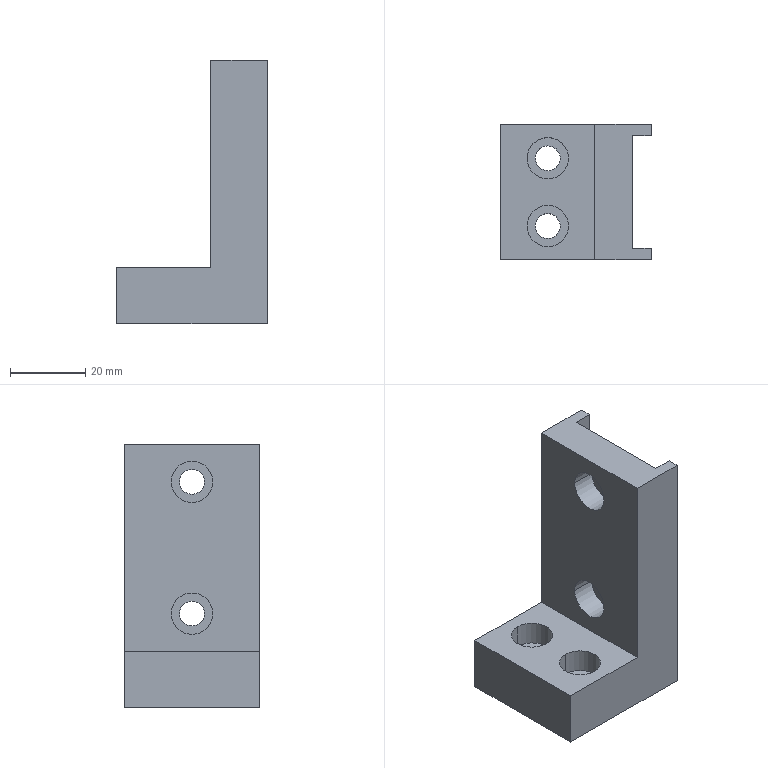Component | SolidWorks | XM-WST05-2008-2 | 1 solid | 32 faces | box 40 x 36 x 70 mm | volume 37532 mm3 | cylinder 16 | plane 16 | commonest cylinder face diameters 11 x8 6.6 x8
build123d program:
from build123d import *

# Parameters (mm, degrees)
BOSS_EXTRUDE1_DEPTH                             = 36
SKETCH2_W                                       = 10
SKETCH2_H                                       = 30
CUT_EXTRUDE1_DEPTH                              = 89.295
M6_HEX_SOCKET_HEAD_CAP_SCREW_CBORE1_D           = 6.6
M6_HEX_SOCKET_HEAD_CAP_SCREW_CBORE1_CBORE_D     = 11
M6_HEX_SOCKET_HEAD_CAP_SCREW_CBORE1_CBORE_DEPTH = 6.4
M6_HEX_SOCKET_HEAD_CAP_SCREW_CBORE2_D           = 6.6
M6_HEX_SOCKET_HEAD_CAP_SCREW_CBORE2_CBORE_D     = 11
M6_HEX_SOCKET_HEAD_CAP_SCREW_CBORE2_CBORE_DEPTH = 6.4


with BuildPart() as part:
    # Sketch1 → Boss-Extrude1 (new body)
    with BuildSketch(Plane.XY):
        Polygon((0, 0), (40, 0), (40, 15), (15, 15), (15, 70), (0, 70), align=None)
    extrude(amount=BOSS_EXTRUDE1_DEPTH)

    # Sketch2 → Cut-Extrude1 (cut, through all)
    with BuildSketch(Plane(origin=(0, 70, 0), x_dir=(1, 0, 0), z_dir=(0, 1, 0))):
        with Locations((0, -18)):
            Rectangle(SKETCH2_W, SKETCH2_H)
    extrude(amount=-CUT_EXTRUDE1_DEPTH, mode=Mode.SUBTRACT)

    # M6 Hex Socket Head Cap Screw CBORE1 (through all)
    with Locations(Plane(origin=(15, 0, 0), x_dir=(0, 0, -1), z_dir=(1, 0, 0))):
        with Locations((-18, 60), (-18, 25)):
            CounterBoreHole(M6_HEX_SOCKET_HEAD_CAP_SCREW_CBORE1_D / 2, M6_HEX_SOCKET_HEAD_CAP_SCREW_CBORE1_CBORE_D / 2, M6_HEX_SOCKET_HEAD_CAP_SCREW_CBORE1_CBORE_DEPTH)

    # M6 Hex Socket Head Cap Screw CBORE2 (through all)
    with Locations(Plane(origin=(0, 15, 0), x_dir=(-1, 0, 0), z_dir=(0, 1, 0))):
        with Locations((-27.5, 9), (-27.5, 27)):
            CounterBoreHole(M6_HEX_SOCKET_HEAD_CAP_SCREW_CBORE2_D / 2, M6_HEX_SOCKET_HEAD_CAP_SCREW_CBORE2_CBORE_D / 2, M6_HEX_SOCKET_HEAD_CAP_SCREW_CBORE2_CBORE_DEPTH)


solid = part.part

# Placed as in the assembly
solid = solid.moved(Location((-164.071, 30.669, 100.899), (-90, 0, 180)))
STEP:
#1=COLOUR_RGB('',0.7922,0.8196,0.9333);
#2=FILL_AREA_STYLE_COLOUR('',#1);
#3=FILL_AREA_STYLE('',(#2));
#4=SURFACE_STYLE_FILL_AREA(#3);
#5=SURFACE_SIDE_STYLE('',(#4));
#6=SURFACE_STYLE_USAGE(.BOTH.,#5);
#7=PRESENTATION_STYLE_ASSIGNMENT((#6));
#8=CARTESIAN_POINT('',(-7.542,1.345,4.311));
#9=VERTEX_POINT('',#8);
#10=CARTESIAN_POINT('',(-7.542,1.778,4.311));
#11=VERTEX_POINT('',#10);
#12=CARTESIAN_POINT('',(-7.542,1.562,4.311));
#13=DIRECTION('',(0.,-0.,1.));
#14=DIRECTION('',(0.,1.,0.));
#15=AXIS2_PLACEMENT_3D('',#12,#13,#14);
#16=CIRCLE('',#15,0.2165);
#17=EDGE_CURVE('',#9,#11,#16,.T.);
#18=ORIENTED_EDGE('',*,*,#17,.F.);
#19=CARTESIAN_POINT('',(-7.542,1.345,4.563));
#20=VERTEX_POINT('',#19);
#21=CARTESIAN_POINT('',(-7.542,1.345,4.563));
#22=DIRECTION('',(0.,-0.,1.));
#23=VECTOR('',#22,39.37);
#24=LINE('',#21,#23);
#25=EDGE_CURVE('',#9,#20,#24,.T.);
#26=ORIENTED_EDGE('',*,*,#25,.T.);
#27=CARTESIAN_POINT('',(-7.542,1.778,4.563));
#28=VERTEX_POINT('',#27);
#29=CARTESIAN_POINT('',(-7.542,1.562,4.563));
#30=DIRECTION('',(0.,-0.,1.));
#31=DIRECTION('',(0.,1.,0.));
#32=AXIS2_PLACEMENT_3D('',#29,#30,#31);
#33=CIRCLE('',#32,0.2165);
#34=EDGE_CURVE('',#20,#28,#33,.T.);
#35=ORIENTED_EDGE('',*,*,#34,.T.);
#36=CARTESIAN_POINT('',(-7.542,1.778,4.563));
#37=DIRECTION('',(0.,-0.,1.));
#38=VECTOR('',#37,39.37);
#39=LINE('',#36,#38);
#40=EDGE_CURVE('',#11,#28,#39,.T.);
#41=ORIENTED_EDGE('',*,*,#40,.F.);
#42=EDGE_LOOP('',(#18,#26,#35,#41));
#43=FACE_OUTER_BOUND('',#42,.T.);
#44=CARTESIAN_POINT('',(-7.542,1.562,4.563));
#45=DIRECTION('',(0.,-0.,1.));
#46=DIRECTION('',(0.,1.,0.));
#47=AXIS2_PLACEMENT_3D('',#44,#45,#46);
#48=CYLINDRICAL_SURFACE('',#47,0.2165);
#49=ADVANCED_FACE('',(#43),#48,.F.);
#50=CARTESIAN_POINT('',(-7.542,1.432,3.972));
#51=VERTEX_POINT('',#50);
#52=CARTESIAN_POINT('',(-7.542,1.692,3.972));
#53=VERTEX_POINT('',#52);
#54=CARTESIAN_POINT('',(-7.542,1.562,3.972));
#55=DIRECTION('',(0.,-0.,1.));
#56=DIRECTION('',(0.,1.,0.));
#57=AXIS2_PLACEMENT_3D('',#54,#55,#56);
#58=CIRCLE('',#57,0.1299);
#59=EDGE_CURVE('',#51,#53,#58,.T.);
#60=ORIENTED_EDGE('',*,*,#59,.F.);
#61=CARTESIAN_POINT('',(-7.542,1.432,4.311));
#62=VERTEX_POINT('',#61);
#63=CARTESIAN_POINT('',(-7.542,1.432,4.563));
#64=DIRECTION('',(0.,-0.,1.));
#65=VECTOR('',#64,39.37);
#66=LINE('',#63,#65);
#67=EDGE_CURVE('',#51,#62,#66,.T.);
#68=ORIENTED_EDGE('',*,*,#67,.T.);
#69=CARTESIAN_POINT('',(-7.542,1.692,4.311));
#70=VERTEX_POINT('',#69);
#71=CARTESIAN_POINT('',(-7.542,1.562,4.311));
#72=DIRECTION('',(0.,-0.,1.));
#73=DIRECTION('',(0.,1.,0.));
#74=AXIS2_PLACEMENT_3D('',#71,#72,#73);
#75=CIRCLE('',#74,0.1299);
#76=EDGE_CURVE('',#62,#70,#75,.T.);
#77=ORIENTED_EDGE('',*,*,#76,.T.);
#78=CARTESIAN_POINT('',(-7.542,1.692,4.563));
#79=DIRECTION('',(0.,-0.,1.));
#80=VECTOR('',#79,39.37);
#81=LINE('',#78,#80);
#82=EDGE_CURVE('',#53,#70,#81,.T.);
#83=ORIENTED_EDGE('',*,*,#82,.F.);
#84=EDGE_LOOP('',(#60,#68,#77,#83));
#85=FACE_OUTER_BOUND('',#84,.T.);
#86=CARTESIAN_POINT('',(-7.542,1.562,4.563));
#87=DIRECTION('',(0.,-0.,1.));
#88=DIRECTION('',(0.,1.,0.));
#89=AXIS2_PLACEMENT_3D('',#86,#87,#88);
#90=CYLINDRICAL_SURFACE('',#89,0.1299);
#91=ADVANCED_FACE('',(#85),#90,.F.);
#92=CARTESIAN_POINT('',(-7.542,2.054,4.311));
#93=VERTEX_POINT('',#92);
#94=CARTESIAN_POINT('',(-7.542,2.487,4.311));
#95=VERTEX_POINT('',#94);
#96=CARTESIAN_POINT('',(-7.542,2.27,4.311));
#97=DIRECTION('',(0.,-0.,1.));
#98=DIRECTION('',(0.,1.,0.));
#99=AXIS2_PLACEMENT_3D('',#96,#97,#98);
#100=CIRCLE('',#99,0.2165);
#101=EDGE_CURVE('',#93,#95,#100,.T.);
#102=ORIENTED_EDGE('',*,*,#101,.F.);
#103=CARTESIAN_POINT('',(-7.542,2.054,4.563));
#104=VERTEX_POINT('',#103);
#105=CARTESIAN_POINT('',(-7.542,2.054,4.563));
#106=DIRECTION('',(0.,-0.,1.));
#107=VECTOR('',#106,39.37);
#108=LINE('',#105,#107);
#109=EDGE_CURVE('',#93,#104,#108,.T.);
#110=ORIENTED_EDGE('',*,*,#109,.T.);
#111=CARTESIAN_POINT('',(-7.542,2.487,4.563));
#112=VERTEX_POINT('',#111);
#113=CARTESIAN_POINT('',(-7.542,2.27,4.563));
#114=DIRECTION('',(0.,-0.,1.));
#115=DIRECTION('',(0.,1.,0.));
#116=AXIS2_PLACEMENT_3D('',#113,#114,#115);
#117=CIRCLE('',#116,0.2165);
#118=EDGE_CURVE('',#104,#112,#117,.T.);
#119=ORIENTED_EDGE('',*,*,#118,.T.);
#120=CARTESIAN_POINT('',(-7.542,2.487,4.563));
#121=DIRECTION('',(0.,-0.,1.));
#122=VECTOR('',#121,39.37);
#123=LINE('',#120,#122);
#124=EDGE_CURVE('',#95,#112,#123,.T.);
#125=ORIENTED_EDGE('',*,*,#124,.F.);
#126=EDGE_LOOP('',(#102,#110,#119,#125));
#127=FACE_OUTER_BOUND('',#126,.T.);
#128=CARTESIAN_POINT('',(-7.542,2.27,4.563));
#129=DIRECTION('',(0.,-0.,1.));
#130=DIRECTION('',(0.,1.,0.));
#131=AXIS2_PLACEMENT_3D('',#128,#129,#130);
#132=CYLINDRICAL_SURFACE('',#131,0.2165);
#133=ADVANCED_FACE('',(#127),#132,.F.);
#134=CARTESIAN_POINT('',(-7.542,2.141,3.972));
#135=VERTEX_POINT('',#134);
#136=CARTESIAN_POINT('',(-7.542,2.4,3.972));
#137=VERTEX_POINT('',#136);
#138=CARTESIAN_POINT('',(-7.542,2.27,3.972));
#139=DIRECTION('',(0.,-0.,1.));
#140=DIRECTION('',(0.,1.,0.));
#141=AXIS2_PLACEMENT_3D('',#138,#139,#140);
#142=CIRCLE('',#141,0.1299);
#143=EDGE_CURVE('',#135,#137,#142,.T.);
#144=ORIENTED_EDGE('',*,*,#143,.F.);
#145=CARTESIAN_POINT('',(-7.542,2.141,4.311));
#146=VERTEX_POINT('',#145);
#147=CARTESIAN_POINT('',(-7.542,2.141,4.563));
#148=DIRECTION('',(0.,-0.,1.));
#149=VECTOR('',#148,39.37);
#150=LINE('',#147,#149);
#151=EDGE_CURVE('',#135,#146,#150,.T.);
#152=ORIENTED_EDGE('',*,*,#151,.T.);
#153=CARTESIAN_POINT('',(-7.542,2.4,4.311));
#154=VERTEX_POINT('',#153);
#155=CARTESIAN_POINT('',(-7.542,2.27,4.311));
#156=DIRECTION('',(0.,-0.,1.));
#157=DIRECTION('',(0.,1.,0.));
#158=AXIS2_PLACEMENT_3D('',#155,#156,#157);
#159=CIRCLE('',#158,0.1299);
#160=EDGE_CURVE('',#146,#154,#159,.T.);
#161=ORIENTED_EDGE('',*,*,#160,.T.);
#162=CARTESIAN_POINT('',(-7.542,2.4,4.563));
#163=DIRECTION('',(0.,-0.,1.));
#164=VECTOR('',#163,39.37);
#165=LINE('',#162,#164);
#166=EDGE_CURVE('',#137,#154,#165,.T.);
#167=ORIENTED_EDGE('',*,*,#166,.F.);
#168=EDGE_LOOP('',(#144,#152,#161,#167));
#169=FACE_OUTER_BOUND('',#168,.T.);
#170=CARTESIAN_POINT('',(-7.542,2.27,4.563));
#171=DIRECTION('',(0.,-0.,1.));
#172=DIRECTION('',(0.,1.,0.));
#173=AXIS2_PLACEMENT_3D('',#170,#171,#172);
#174=CYLINDRICAL_SURFACE('',#173,0.1299);
#175=ADVANCED_FACE('',(#169),#174,.F.);
#176=CARTESIAN_POINT('',(-6.798,2.133,6.335));
#177=VERTEX_POINT('',#176);
#178=CARTESIAN_POINT('',(-6.798,1.7,6.335));
#179=VERTEX_POINT('',#178);
#180=CARTESIAN_POINT('',(-6.798,1.916,6.335));
#181=DIRECTION('',(-1.,0.,0.));
#182=DIRECTION('',(0.,-1.,0.));
#183=AXIS2_PLACEMENT_3D('',#180,#181,#182);
#184=CIRCLE('',#183,0.2165);
#185=EDGE_CURVE('',#177,#179,#184,.T.);
#186=ORIENTED_EDGE('',*,*,#185,.F.);
#187=CARTESIAN_POINT('',(-7.05,2.133,6.335));
#188=VERTEX_POINT('',#187);
#189=CARTESIAN_POINT('',(-7.05,2.133,6.335));
#190=DIRECTION('',(-1.,0.,0.));
#191=VECTOR('',#190,39.37);
#192=LINE('',#189,#191);
#193=EDGE_CURVE('',#177,#188,#192,.T.);
#194=ORIENTED_EDGE('',*,*,#193,.T.);
#195=CARTESIAN_POINT('',(-7.05,1.7,6.335));
#196=VERTEX_POINT('',#195);
#197=CARTESIAN_POINT('',(-7.05,1.916,6.335));
#198=DIRECTION('',(-1.,0.,0.));
#199=DIRECTION('',(0.,-1.,0.));
#200=AXIS2_PLACEMENT_3D('',#197,#198,#199);
#201=CIRCLE('',#200,0.2165);
#202=EDGE_CURVE('',#188,#196,#201,.T.);
#203=ORIENTED_EDGE('',*,*,#202,.T.);
#204=CARTESIAN_POINT('',(-7.05,1.7,6.335));
#205=DIRECTION('',(-1.,0.,0.));
#206=VECTOR('',#205,39.37);
#207=LINE('',#204,#206);
#208=EDGE_CURVE('',#179,#196,#207,.T.);
#209=ORIENTED_EDGE('',*,*,#208,.F.);
#210=EDGE_LOOP('',(#186,#194,#203,#209));
#211=FACE_OUTER_BOUND('',#210,.T.);
#212=CARTESIAN_POINT('',(-7.05,1.916,6.335));
#213=DIRECTION('',(-1.,0.,0.));
#214=DIRECTION('',(0.,-1.,0.));
#215=AXIS2_PLACEMENT_3D('',#212,#213,#214);
#216=CYLINDRICAL_SURFACE('',#215,0.2165);
#217=ADVANCED_FACE('',(#211),#216,.F.);
#218=CARTESIAN_POINT('',(-6.656,2.046,6.335));
#219=VERTEX_POINT('',#218);
#220=CARTESIAN_POINT('',(-6.656,1.786,6.335));
#221=VERTEX_POINT('',#220);
#222=CARTESIAN_POINT('',(-6.656,1.916,6.335));
#223=DIRECTION('',(-1.,0.,0.));
#224=DIRECTION('',(0.,-1.,0.));
#225=AXIS2_PLACEMENT_3D('',#222,#223,#224);
#226=CIRCLE('',#225,0.1299);
#227=EDGE_CURVE('',#219,#221,#226,.T.);
#228=ORIENTED_EDGE('',*,*,#227,.F.);
#229=CARTESIAN_POINT('',(-6.798,2.046,6.335));
#230=VERTEX_POINT('',#229);
#231=CARTESIAN_POINT('',(-7.05,2.046,6.335));
#232=DIRECTION('',(-1.,0.,0.));
#233=VECTOR('',#232,39.37);
#234=LINE('',#231,#233);
#235=EDGE_CURVE('',#219,#230,#234,.T.);
#236=ORIENTED_EDGE('',*,*,#235,.T.);
#237=CARTESIAN_POINT('',(-6.798,1.786,6.335));
#238=VERTEX_POINT('',#237);
#239=CARTESIAN_POINT('',(-6.798,1.916,6.335));
#240=DIRECTION('',(-1.,0.,0.));
#241=DIRECTION('',(0.,-1.,0.));
#242=AXIS2_PLACEMENT_3D('',#239,#240,#241);
#243=CIRCLE('',#242,0.1299);
#244=EDGE_CURVE('',#230,#238,#243,.T.);
#245=ORIENTED_EDGE('',*,*,#244,.T.);
#246=CARTESIAN_POINT('',(-7.05,1.786,6.335));
#247=DIRECTION('',(-1.,0.,0.));
#248=VECTOR('',#247,39.37);
#249=LINE('',#246,#248);
#250=EDGE_CURVE('',#221,#238,#249,.T.);
#251=ORIENTED_EDGE('',*,*,#250,.F.);
#252=EDGE_LOOP('',(#228,#236,#245,#251));
#253=FACE_OUTER_BOUND('',#252,.T.);
#254=CARTESIAN_POINT('',(-7.05,1.916,6.335));
#255=DIRECTION('',(-1.,0.,0.));
#256=DIRECTION('',(0.,-1.,0.));
#257=AXIS2_PLACEMENT_3D('',#254,#255,#256);
#258=CYLINDRICAL_SURFACE('',#257,0.1299);
#259=ADVANCED_FACE('',(#253),#258,.F.);
#260=CARTESIAN_POINT('',(-6.798,2.133,4.957));
#261=VERTEX_POINT('',#260);
#262=CARTESIAN_POINT('',(-6.798,1.7,4.957));
#263=VERTEX_POINT('',#262);
#264=CARTESIAN_POINT('',(-6.798,1.916,4.957));
#265=DIRECTION('',(-1.,0.,0.));
#266=DIRECTION('',(0.,-1.,0.));
#267=AXIS2_PLACEMENT_3D('',#264,#265,#266);
#268=CIRCLE('',#267,0.2165);
#269=EDGE_CURVE('',#261,#263,#268,.T.);
#270=ORIENTED_EDGE('',*,*,#269,.F.);
#271=CARTESIAN_POINT('',(-7.05,2.133,4.957));
#272=VERTEX_POINT('',#271);
#273=CARTESIAN_POINT('',(-7.05,2.133,4.957));
#274=DIRECTION('',(-1.,0.,0.));
#275=VECTOR('',#274,39.37);
#276=LINE('',#273,#275);
#277=EDGE_CURVE('',#261,#272,#276,.T.);
#278=ORIENTED_EDGE('',*,*,#277,.T.);
#279=CARTESIAN_POINT('',(-7.05,1.7,4.957));
#280=VERTEX_POINT('',#279);
#281=CARTESIAN_POINT('',(-7.05,1.916,4.957));
#282=DIRECTION('',(-1.,0.,0.));
#283=DIRECTION('',(0.,-1.,0.));
#284=AXIS2_PLACEMENT_3D('',#281,#282,#283);
#285=CIRCLE('',#284,0.2165);
#286=EDGE_CURVE('',#272,#280,#285,.T.);
#287=ORIENTED_EDGE('',*,*,#286,.T.);
#288=CARTESIAN_POINT('',(-7.05,1.7,4.957));
#289=DIRECTION('',(-1.,0.,0.));
#290=VECTOR('',#289,39.37);
#291=LINE('',#288,#290);
#292=EDGE_CURVE('',#263,#280,#291,.T.);
#293=ORIENTED_EDGE('',*,*,#292,.F.);
#294=EDGE_LOOP('',(#270,#278,#287,#293));
#295=FACE_OUTER_BOUND('',#294,.T.);
#296=CARTESIAN_POINT('',(-7.05,1.916,4.957));
#297=DIRECTION('',(-1.,0.,0.));
#298=DIRECTION('',(0.,-1.,0.));
#299=AXIS2_PLACEMENT_3D('',#296,#297,#298);
#300=CYLINDRICAL_SURFACE('',#299,0.2165);
#301=ADVANCED_FACE('',(#295),#300,.F.);
#302=CARTESIAN_POINT('',(-6.656,2.046,4.957));
#303=VERTEX_POINT('',#302);
#304=CARTESIAN_POINT('',(-6.656,1.786,4.957));
#305=VERTEX_POINT('',#304);
#306=CARTESIAN_POINT('',(-6.656,1.916,4.957));
#307=DIRECTION('',(-1.,0.,0.));
#308=DIRECTION('',(0.,-1.,0.));
#309=AXIS2_PLACEMENT_3D('',#306,#307,#308);
#310=CIRCLE('',#309,0.1299);
#311=EDGE_CURVE('',#303,#305,#310,.T.);
#312=ORIENTED_EDGE('',*,*,#311,.F.);
#313=CARTESIAN_POINT('',(-6.798,2.046,4.957));
#314=VERTEX_POINT('',#313);
#315=CARTESIAN_POINT('',(-7.05,2.046,4.957));
#316=DIRECTION('',(-1.,0.,0.));
#317=VECTOR('',#316,39.37);
#318=LINE('',#315,#317);
#319=EDGE_CURVE('',#303,#314,#318,.T.);
#320=ORIENTED_EDGE('',*,*,#319,.T.);
#321=CARTESIAN_POINT('',(-6.798,1.786,4.957));
#322=VERTEX_POINT('',#321);
#323=CARTESIAN_POINT('',(-6.798,1.916,4.957));
#324=DIRECTION('',(-1.,0.,0.));
#325=DIRECTION('',(0.,-1.,0.));
#326=AXIS2_PLACEMENT_3D('',#323,#324,#325);
#327=CIRCLE('',#326,0.1299);
#328=EDGE_CURVE('',#314,#322,#327,.T.);
#329=ORIENTED_EDGE('',*,*,#328,.T.);
#330=CARTESIAN_POINT('',(-7.05,1.786,4.957));
#331=DIRECTION('',(-1.,0.,0.));
#332=VECTOR('',#331,39.37);
#333=LINE('',#330,#332);
#334=EDGE_CURVE('',#305,#322,#333,.T.);
#335=ORIENTED_EDGE('',*,*,#334,.F.);
#336=EDGE_LOOP('',(#312,#320,#329,#335));
#337=FACE_OUTER_BOUND('',#336,.T.);
#338=CARTESIAN_POINT('',(-7.05,1.916,4.957));
#339=DIRECTION('',(-1.,0.,0.));
#340=DIRECTION('',(0.,-1.,0.));
#341=AXIS2_PLACEMENT_3D('',#338,#339,#340);
#342=CYLINDRICAL_SURFACE('',#341,0.1299);
#343=ADVANCED_FACE('',(#337),#342,.F.);
#344=CARTESIAN_POINT('',(-6.459,2.625,6.728));
#345=VERTEX_POINT('',#344);
#346=CARTESIAN_POINT('',(-6.459,2.507,6.728));
#347=VERTEX_POINT('',#346);
#348=CARTESIAN_POINT('',(-6.459,2.625,6.728));
#349=DIRECTION('',(-0.,-1.,-0.));
#350=VECTOR('',#349,39.37);
#351=LINE('',#348,#350);
#352=EDGE_CURVE('',#345,#347,#351,.T.);
#353=ORIENTED_EDGE('',*,*,#352,.T.);
#354=CARTESIAN_POINT('',(-6.459,2.507,3.972));
#355=VERTEX_POINT('',#354);
#356=CARTESIAN_POINT('',(-6.459,2.507,6.728));
#357=DIRECTION('',(0.,0.,-1.));
#358=VECTOR('',#357,39.37);
#359=LINE('',#356,#358);
#360=EDGE_CURVE('',#347,#355,#359,.T.);
#361=ORIENTED_EDGE('',*,*,#360,.T.);
#362=CARTESIAN_POINT('',(-6.459,2.625,3.972));
#363=VERTEX_POINT('',#362);
#364=CARTESIAN_POINT('',(-6.459,2.625,3.972));
#365=DIRECTION('',(-0.,-1.,-0.));
#366=VECTOR('',#365,39.37);
#367=LINE('',#364,#366);
#368=EDGE_CURVE('',#363,#355,#367,.T.);
#369=ORIENTED_EDGE('',*,*,#368,.F.);
#370=CARTESIAN_POINT('',(-6.459,2.625,6.728));
#371=DIRECTION('',(0.,0.,-1.));
#372=VECTOR('',#371,39.37);
#373=LINE('',#370,#372);
#374=EDGE_CURVE('',#345,#363,#373,.T.);
#375=ORIENTED_EDGE('',*,*,#374,.F.);
#376=EDGE_LOOP('',(#353,#361,#369,#375));
#377=FACE_OUTER_BOUND('',#376,.T.);
#378=CARTESIAN_POINT('',(-6.459,2.625,6.728));
#379=DIRECTION('',(-1.,0.,-0.));
#380=DIRECTION('',(-0.,-0.,1.));
#381=AXIS2_PLACEMENT_3D('',#378,#379,#380);
#382=PLANE('',#381);
#383=ADVANCED_FACE('',(#377),#382,.F.);
#384=CARTESIAN_POINT('',(-6.459,1.326,3.972));
#385=VERTEX_POINT('',#384);
#386=CARTESIAN_POINT('',(-6.459,1.207,3.972));
#387=VERTEX_POINT('',#386);
#388=CARTESIAN_POINT('',(-6.459,2.625,3.972));
#389=DIRECTION('',(-0.,-1.,-0.));
#390=VECTOR('',#389,39.37);
#391=LINE('',#388,#390);
#392=EDGE_CURVE('',#385,#387,#391,.T.);
#393=ORIENTED_EDGE('',*,*,#392,.F.);
#394=CARTESIAN_POINT('',(-6.459,1.326,6.728));
#395=VERTEX_POINT('',#394);
#396=CARTESIAN_POINT('',(-6.459,1.326,6.728));
#397=DIRECTION('',(-0.,-0.,1.));
#398=VECTOR('',#397,39.37);
#399=LINE('',#396,#398);
#400=EDGE_CURVE('',#385,#395,#399,.T.);
#401=ORIENTED_EDGE('',*,*,#400,.T.);
#402=CARTESIAN_POINT('',(-6.459,1.207,6.728));
#403=VERTEX_POINT('',#402);
#404=CARTESIAN_POINT('',(-6.459,2.625,6.728));
#405=DIRECTION('',(-0.,-1.,-0.));
#406=VECTOR('',#405,39.37);
#407=LINE('',#404,#406);
#408=EDGE_CURVE('',#395,#403,#407,.T.);
#409=ORIENTED_EDGE('',*,*,#408,.T.);
#410=CARTESIAN_POINT('',(-6.459,1.207,6.728));
#411=DIRECTION('',(0.,0.,-1.));
#412=VECTOR('',#411,39.37);
#413=LINE('',#410,#412);
#414=EDGE_CURVE('',#403,#387,#413,.T.);
#415=ORIENTED_EDGE('',*,*,#414,.T.);
#416=EDGE_LOOP('',(#393,#401,#409,#415));
#417=FACE_OUTER_BOUND('',#416,.T.);
#418=CARTESIAN_POINT('',(-6.459,2.625,6.728));
#419=DIRECTION('',(-1.,0.,-0.));
#420=DIRECTION('',(-0.,-0.,1.));
#421=AXIS2_PLACEMENT_3D('',#418,#419,#420);
#422=PLANE('',#421);
#423=ADVANCED_FACE('',(#417),#422,.F.);
#424=CARTESIAN_POINT('',(-7.542,1.562,3.972));
#425=DIRECTION('',(0.,-0.,1.));
#426=DIRECTION('',(0.,1.,0.));
#427=AXIS2_PLACEMENT_3D('',#424,#425,#426);
#428=CIRCLE('',#427,0.1299);
#429=EDGE_CURVE('',#53,#51,#428,.T.);
#430=ORIENTED_EDGE('',*,*,#429,.T.);
#431=ORIENTED_EDGE('',*,*,#59,.T.);
#432=EDGE_LOOP('',(#430,#431));
#433=FACE_BOUND('',#432,.T.);
#434=CARTESIAN_POINT('',(-7.542,2.27,3.972));
#435=DIRECTION('',(0.,-0.,1.));
#436=DIRECTION('',(0.,1.,0.));
#437=AXIS2_PLACEMENT_3D('',#434,#435,#436);
#438=CIRCLE('',#437,0.1299);
#439=EDGE_CURVE('',#137,#135,#438,.T.);
#440=ORIENTED_EDGE('',*,*,#439,.T.);
#441=ORIENTED_EDGE('',*,*,#143,.T.);
#442=EDGE_LOOP('',(#440,#441));
#443=FACE_BOUND('',#442,.T.);
#444=ORIENTED_EDGE('',*,*,#368,.T.);
#445=CARTESIAN_POINT('',(-6.656,2.507,3.972));
#446=VERTEX_POINT('',#445);
#447=CARTESIAN_POINT('',(-6.263,2.507,3.972));
#448=DIRECTION('',(-1.,0.,0.));
#449=VECTOR('',#448,39.37);
#450=LINE('',#447,#449);
#451=EDGE_CURVE('',#355,#446,#450,.T.);
#452=ORIENTED_EDGE('',*,*,#451,.T.);
#453=CARTESIAN_POINT('',(-6.656,1.326,3.972));
#454=VERTEX_POINT('',#453);
#455=CARTESIAN_POINT('',(-6.656,1.326,3.972));
#456=DIRECTION('',(-0.,-1.,-0.));
#457=VECTOR('',#456,39.37);
#458=LINE('',#455,#457);
#459=EDGE_CURVE('',#446,#454,#458,.T.);
#460=ORIENTED_EDGE('',*,*,#459,.T.);
#461=CARTESIAN_POINT('',(-6.263,1.326,3.972));
#462=DIRECTION('',(1.,-0.,-0.));
#463=VECTOR('',#462,39.37);
#464=LINE('',#461,#463);
#465=EDGE_CURVE('',#454,#385,#464,.T.);
#466=ORIENTED_EDGE('',*,*,#465,.T.);
#467=ORIENTED_EDGE('',*,*,#392,.T.);
#468=CARTESIAN_POINT('',(-8.034,1.207,3.972));
#469=VERTEX_POINT('',#468);
#470=CARTESIAN_POINT('',(-6.459,1.207,3.972));
#471=DIRECTION('',(-1.,0.,0.));
#472=VECTOR('',#471,39.37);
#473=LINE('',#470,#472);
#474=EDGE_CURVE('',#387,#469,#473,.T.);
#475=ORIENTED_EDGE('',*,*,#474,.T.);
#476=CARTESIAN_POINT('',(-8.034,2.625,3.972));
#477=VERTEX_POINT('',#476);
#478=CARTESIAN_POINT('',(-8.034,2.625,3.972));
#479=DIRECTION('',(-0.,-1.,-0.));
#480=VECTOR('',#479,39.37);
#481=LINE('',#478,#480);
#482=EDGE_CURVE('',#477,#469,#481,.T.);
#483=ORIENTED_EDGE('',*,*,#482,.F.);
#484=CARTESIAN_POINT('',(-6.459,2.625,3.972));
#485=DIRECTION('',(-1.,0.,0.));
#486=VECTOR('',#485,39.37);
#487=LINE('',#484,#486);
#488=EDGE_CURVE('',#363,#477,#487,.T.);
#489=ORIENTED_EDGE('',*,*,#488,.F.);
#490=EDGE_LOOP('',(#444,#452,#460,#466,#467,#475,#483,#489));
#491=FACE_OUTER_BOUND('',#490,.T.);
#492=CARTESIAN_POINT('',(-6.459,2.625,3.972));
#493=DIRECTION('',(0.,-0.,1.));
#494=DIRECTION('',(0.,1.,0.));
#495=AXIS2_PLACEMENT_3D('',#492,#493,#494);
#496=PLANE('',#495);
#497=ADVANCED_FACE('',(#433,#443,#491),#496,.F.);
#498=CARTESIAN_POINT('',(-8.034,1.207,4.563));
#499=VERTEX_POINT('',#498);
#500=CARTESIAN_POINT('',(-8.034,1.207,3.972));
#501=DIRECTION('',(0.,-0.,1.));
#502=VECTOR('',#501,39.37);
#503=LINE('',#500,#502);
#504=EDGE_CURVE('',#469,#499,#503,.T.);
#505=ORIENTED_EDGE('',*,*,#504,.T.);
#506=CARTESIAN_POINT('',(-8.034,2.625,4.563));
#507=VERTEX_POINT('',#506);
#508=CARTESIAN_POINT('',(-8.034,2.625,4.563));
#509=DIRECTION('',(-0.,-1.,-0.));
#510=VECTOR('',#509,39.37);
#511=LINE('',#508,#510);
#512=EDGE_CURVE('',#507,#499,#511,.T.);
#513=ORIENTED_EDGE('',*,*,#512,.F.);
#514=CARTESIAN_POINT('',(-8.034,2.625,3.972));
#515=DIRECTION('',(0.,-0.,1.));
#516=VECTOR('',#515,39.37);
#517=LINE('',#514,#516);
#518=EDGE_CURVE('',#477,#507,#517,.T.);
#519=ORIENTED_EDGE('',*,*,#518,.F.);
#520=ORIENTED_EDGE('',*,*,#482,.T.);
#521=EDGE_LOOP('',(#505,#513,#519,#520));
#522=FACE_OUTER_BOUND('',#521,.T.);
#523=CARTESIAN_POINT('',(-8.034,2.625,3.972));
#524=DIRECTION('',(1.,-0.,-0.));
#525=DIRECTION('',(0.,1.,0.));
#526=AXIS2_PLACEMENT_3D('',#523,#524,#525);
#527=PLANE('',#526);
#528=ADVANCED_FACE('',(#522),#527,.F.);
#529=CARTESIAN_POINT('',(-7.542,1.562,4.563));
#530=DIRECTION('',(0.,-0.,1.));
#531=DIRECTION('',(0.,1.,0.));
#532=AXIS2_PLACEMENT_3D('',#529,#530,#531);
#533=CIRCLE('',#532,0.2165);
#534=EDGE_CURVE('',#28,#20,#533,.T.);
#535=ORIENTED_EDGE('',*,*,#534,.F.);
#536=ORIENTED_EDGE('',*,*,#34,.F.);
#537=EDGE_LOOP('',(#535,#536));
#538=FACE_BOUND('',#537,.T.);
#539=CARTESIAN_POINT('',(-7.542,2.27,4.563));
#540=DIRECTION('',(0.,-0.,1.));
#541=DIRECTION('',(0.,1.,0.));
#542=AXIS2_PLACEMENT_3D('',#539,#540,#541);
#543=CIRCLE('',#542,0.2165);
#544=EDGE_CURVE('',#112,#104,#543,.T.);
#545=ORIENTED_EDGE('',*,*,#544,.F.);
#546=ORIENTED_EDGE('',*,*,#118,.F.);
#547=EDGE_LOOP('',(#545,#546));
#548=FACE_BOUND('',#547,.T.);
#549=CARTESIAN_POINT('',(-7.05,1.207,4.563));
#550=VERTEX_POINT('',#549);
#551=CARTESIAN_POINT('',(-8.034,1.207,4.563));
#552=DIRECTION('',(1.,-0.,-0.));
#553=VECTOR('',#552,39.37);
#554=LINE('',#551,#553);
#555=EDGE_CURVE('',#499,#550,#554,.T.);
#556=ORIENTED_EDGE('',*,*,#555,.T.);
#557=CARTESIAN_POINT('',(-7.05,2.625,4.563));
#558=VERTEX_POINT('',#557);
#559=CARTESIAN_POINT('',(-7.05,2.625,4.563));
#560=DIRECTION('',(-0.,-1.,-0.));
#561=VECTOR('',#560,39.37);
#562=LINE('',#559,#561);
#563=EDGE_CURVE('',#558,#550,#562,.T.);
#564=ORIENTED_EDGE('',*,*,#563,.F.);
#565=CARTESIAN_POINT('',(-8.034,2.625,4.563));
#566=DIRECTION('',(1.,-0.,-0.));
#567=VECTOR('',#566,39.37);
#568=LINE('',#565,#567);
#569=EDGE_CURVE('',#507,#558,#568,.T.);
#570=ORIENTED_EDGE('',*,*,#569,.F.);
#571=ORIENTED_EDGE('',*,*,#512,.T.);
#572=EDGE_LOOP('',(#556,#564,#570,#571));
#573=FACE_OUTER_BOUND('',#572,.T.);
#574=CARTESIAN_POINT('',(-8.034,2.625,4.563));
#575=DIRECTION('',(-0.,0.,-1.));
#576=DIRECTION('',(-1.,0.,0.));
#577=AXIS2_PLACEMENT_3D('',#574,#575,#576);
#578=PLANE('',#577);
#579=ADVANCED_FACE('',(#538,#548,#573),#578,.F.);
#580=CARTESIAN_POINT('',(-7.05,1.916,6.335));
#581=DIRECTION('',(-1.,0.,0.));
#582=DIRECTION('',(0.,-1.,0.));
#583=AXIS2_PLACEMENT_3D('',#580,#581,#582);
#584=CIRCLE('',#583,0.2165);
#585=EDGE_CURVE('',#196,#188,#584,.T.);
#586=ORIENTED_EDGE('',*,*,#585,.F.);
#587=ORIENTED_EDGE('',*,*,#202,.F.);
#588=EDGE_LOOP('',(#586,#587));
#589=FACE_BOUND('',#588,.T.);
#590=CARTESIAN_POINT('',(-7.05,1.916,4.957));
#591=DIRECTION('',(-1.,0.,0.));
#592=DIRECTION('',(0.,-1.,0.));
#593=AXIS2_PLACEMENT_3D('',#590,#591,#592);
#594=CIRCLE('',#593,0.2165);
#595=EDGE_CURVE('',#280,#272,#594,.T.);
#596=ORIENTED_EDGE('',*,*,#595,.F.);
#597=ORIENTED_EDGE('',*,*,#286,.F.);
#598=EDGE_LOOP('',(#596,#597));
#599=FACE_BOUND('',#598,.T.);
#600=CARTESIAN_POINT('',(-7.05,1.207,6.728));
#601=VERTEX_POINT('',#600);
#602=CARTESIAN_POINT('',(-7.05,1.207,4.563));
#603=DIRECTION('',(-0.,-0.,1.));
#604=VECTOR('',#603,39.37);
#605=LINE('',#602,#604);
#606=EDGE_CURVE('',#550,#601,#605,.T.);
#607=ORIENTED_EDGE('',*,*,#606,.T.);
#608=CARTESIAN_POINT('',(-7.05,2.625,6.728));
#609=VERTEX_POINT('',#608);
#610=CARTESIAN_POINT('',(-7.05,2.625,6.728));
#611=DIRECTION('',(-0.,-1.,-0.));
#612=VECTOR('',#611,39.37);
#613=LINE('',#610,#612);
#614=EDGE_CURVE('',#609,#601,#613,.T.);
#615=ORIENTED_EDGE('',*,*,#614,.F.);
#616=CARTESIAN_POINT('',(-7.05,2.625,4.563));
#617=DIRECTION('',(-0.,-0.,1.));
#618=VECTOR('',#617,39.37);
#619=LINE('',#616,#618);
#620=EDGE_CURVE('',#558,#609,#619,.T.);
#621=ORIENTED_EDGE('',*,*,#620,.F.);
#622=ORIENTED_EDGE('',*,*,#563,.T.);
#623=EDGE_LOOP('',(#607,#615,#621,#622));
#624=FACE_OUTER_BOUND('',#623,.T.);
#625=CARTESIAN_POINT('',(-7.05,2.625,4.563));
#626=DIRECTION('',(1.,-0.,0.));
#627=DIRECTION('',(0.,0.,-1.));
#628=AXIS2_PLACEMENT_3D('',#625,#626,#627);
#629=PLANE('',#628);
#630=ADVANCED_FACE('',(#589,#599,#624),#629,.F.);
#631=CARTESIAN_POINT('',(-6.656,2.507,6.728));
#632=VERTEX_POINT('',#631);
#633=CARTESIAN_POINT('',(-6.656,1.326,6.728));
#634=VERTEX_POINT('',#633);
#635=CARTESIAN_POINT('',(-6.656,1.326,6.728));
#636=DIRECTION('',(-0.,-1.,-0.));
#637=VECTOR('',#636,39.37);
#638=LINE('',#635,#637);
#639=EDGE_CURVE('',#632,#634,#638,.T.);
#640=ORIENTED_EDGE('',*,*,#639,.F.);
#641=CARTESIAN_POINT('',(-7.05,2.507,6.728));
#642=DIRECTION('',(1.,-0.,-0.));
#643=VECTOR('',#642,39.37);
#644=LINE('',#641,#643);
#645=EDGE_CURVE('',#632,#347,#644,.T.);
#646=ORIENTED_EDGE('',*,*,#645,.T.);
#647=ORIENTED_EDGE('',*,*,#352,.F.);
#648=CARTESIAN_POINT('',(-7.05,2.625,6.728));
#649=DIRECTION('',(1.,-0.,-0.));
#650=VECTOR('',#649,39.37);
#651=LINE('',#648,#650);
#652=EDGE_CURVE('',#609,#345,#651,.T.);
#653=ORIENTED_EDGE('',*,*,#652,.F.);
#654=ORIENTED_EDGE('',*,*,#614,.T.);
#655=CARTESIAN_POINT('',(-7.05,1.207,6.728));
#656=DIRECTION('',(1.,-0.,-0.));
#657=VECTOR('',#656,39.37);
#658=LINE('',#655,#657);
#659=EDGE_CURVE('',#601,#403,#658,.T.);
#660=ORIENTED_EDGE('',*,*,#659,.T.);
#661=ORIENTED_EDGE('',*,*,#408,.F.);
#662=CARTESIAN_POINT('',(-6.263,1.326,6.728));
#663=DIRECTION('',(1.,-0.,-0.));
#664=VECTOR('',#663,39.37);
#665=LINE('',#662,#664);
#666=EDGE_CURVE('',#634,#395,#665,.T.);
#667=ORIENTED_EDGE('',*,*,#666,.F.);
#668=EDGE_LOOP('',(#640,#646,#647,#653,#654,#660,#661,#667));
#669=FACE_OUTER_BOUND('',#668,.T.);
#670=CARTESIAN_POINT('',(-7.05,2.625,6.728));
#671=DIRECTION('',(-0.,0.,-1.));
#672=DIRECTION('',(-0.,-1.,-0.));
#673=AXIS2_PLACEMENT_3D('',#670,#671,#672);
#674=PLANE('',#673);
#675=ADVANCED_FACE('',(#669),#674,.F.);
#676=ORIENTED_EDGE('',*,*,#374,.T.);
#677=ORIENTED_EDGE('',*,*,#488,.T.);
#678=ORIENTED_EDGE('',*,*,#518,.T.);
#679=ORIENTED_EDGE('',*,*,#569,.T.);
#680=ORIENTED_EDGE('',*,*,#620,.T.);
#681=ORIENTED_EDGE('',*,*,#652,.T.);
#682=EDGE_LOOP('',(#676,#677,#678,#679,#680,#681));
#683=FACE_OUTER_BOUND('',#682,.T.);
#684=CARTESIAN_POINT('',(-6.459,2.625,3.972));
#685=DIRECTION('',(0.,1.,0.));
#686=DIRECTION('',(-1.,0.,0.));
#687=AXIS2_PLACEMENT_3D('',#684,#685,#686);
#688=PLANE('',#687);
#689=ADVANCED_FACE('',(#683),#688,.T.);
#690=ORIENTED_EDGE('',*,*,#414,.F.);
#691=ORIENTED_EDGE('',*,*,#659,.F.);
#692=ORIENTED_EDGE('',*,*,#606,.F.);
#693=ORIENTED_EDGE('',*,*,#555,.F.);
#694=ORIENTED_EDGE('',*,*,#504,.F.);
#695=ORIENTED_EDGE('',*,*,#474,.F.);
#696=EDGE_LOOP('',(#690,#691,#692,#693,#694,#695));
#697=FACE_OUTER_BOUND('',#696,.T.);
#698=CARTESIAN_POINT('',(-6.459,1.207,3.972));
#699=DIRECTION('',(0.,1.,0.));
#700=DIRECTION('',(-1.,0.,0.));
#701=AXIS2_PLACEMENT_3D('',#698,#699,#700);
#702=PLANE('',#701);
#703=ADVANCED_FACE('',(#697),#702,.F.);
#704=ORIENTED_EDGE('',*,*,#645,.F.);
#705=CARTESIAN_POINT('',(-6.656,2.507,3.972));
#706=DIRECTION('',(0.,-0.,1.));
#707=VECTOR('',#706,39.37);
#708=LINE('',#705,#707);
#709=EDGE_CURVE('',#446,#632,#708,.T.);
#710=ORIENTED_EDGE('',*,*,#709,.F.);
#711=ORIENTED_EDGE('',*,*,#451,.F.);
#712=ORIENTED_EDGE('',*,*,#360,.F.);
#713=EDGE_LOOP('',(#704,#710,#711,#712));
#714=FACE_OUTER_BOUND('',#713,.T.);
#715=CARTESIAN_POINT('',(-6.263,2.507,3.972));
#716=DIRECTION('',(0.,1.,0.));
#717=DIRECTION('',(-1.,0.,0.));
#718=AXIS2_PLACEMENT_3D('',#715,#716,#717);
#719=PLANE('',#718);
#720=ADVANCED_FACE('',(#714),#719,.F.);
#721=ORIENTED_EDGE('',*,*,#465,.F.);
#722=CARTESIAN_POINT('',(-6.656,1.326,3.972));
#723=DIRECTION('',(0.,-0.,1.));
#724=VECTOR('',#723,39.37);
#725=LINE('',#722,#724);
#726=EDGE_CURVE('',#454,#634,#725,.T.);
#727=ORIENTED_EDGE('',*,*,#726,.T.);
#728=ORIENTED_EDGE('',*,*,#666,.T.);
#729=ORIENTED_EDGE('',*,*,#400,.F.);
#730=EDGE_LOOP('',(#721,#727,#728,#729));
#731=FACE_OUTER_BOUND('',#730,.T.);
#732=CARTESIAN_POINT('',(-6.263,1.326,3.972));
#733=DIRECTION('',(-0.,-1.,-0.));
#734=DIRECTION('',(1.,-0.,-0.));
#735=AXIS2_PLACEMENT_3D('',#732,#733,#734);
#736=PLANE('',#735);
#737=ADVANCED_FACE('',(#731),#736,.F.);
#738=CARTESIAN_POINT('',(-6.656,1.916,6.335));
#739=DIRECTION('',(-1.,0.,0.));
#740=DIRECTION('',(0.,-1.,0.));
#741=AXIS2_PLACEMENT_3D('',#738,#739,#740);
#742=CIRCLE('',#741,0.1299);
#743=EDGE_CURVE('',#221,#219,#742,.T.);
#744=ORIENTED_EDGE('',*,*,#743,.T.);
#745=ORIENTED_EDGE('',*,*,#227,.T.);
#746=EDGE_LOOP('',(#744,#745));
#747=FACE_BOUND('',#746,.T.);
#748=CARTESIAN_POINT('',(-6.656,1.916,4.957));
#749=DIRECTION('',(-1.,0.,0.));
#750=DIRECTION('',(0.,-1.,0.));
#751=AXIS2_PLACEMENT_3D('',#748,#749,#750);
#752=CIRCLE('',#751,0.1299);
#753=EDGE_CURVE('',#305,#303,#752,.T.);
#754=ORIENTED_EDGE('',*,*,#753,.T.);
#755=ORIENTED_EDGE('',*,*,#311,.T.);
#756=EDGE_LOOP('',(#754,#755));
#757=FACE_BOUND('',#756,.T.);
#758=ORIENTED_EDGE('',*,*,#639,.T.);
#759=ORIENTED_EDGE('',*,*,#726,.F.);
#760=ORIENTED_EDGE('',*,*,#459,.F.);
#761=ORIENTED_EDGE('',*,*,#709,.T.);
#762=EDGE_LOOP('',(#758,#759,#760,#761));
#763=FACE_OUTER_BOUND('',#762,.T.);
#764=CARTESIAN_POINT('',(-6.656,1.326,3.972));
#765=DIRECTION('',(-1.,0.,0.));
#766=DIRECTION('',(-0.,-1.,-0.));
#767=AXIS2_PLACEMENT_3D('',#764,#765,#766);
#768=PLANE('',#767);
#769=ADVANCED_FACE('',(#747,#757,#763),#768,.F.);
#770=ORIENTED_EDGE('',*,*,#319,.F.);
#771=ORIENTED_EDGE('',*,*,#753,.F.);
#772=ORIENTED_EDGE('',*,*,#334,.T.);
#773=CARTESIAN_POINT('',(-6.798,1.916,4.957));
#774=DIRECTION('',(-1.,0.,0.));
#775=DIRECTION('',(0.,-1.,0.));
#776=AXIS2_PLACEMENT_3D('',#773,#774,#775);
#777=CIRCLE('',#776,0.1299);
#778=EDGE_CURVE('',#322,#314,#777,.T.);
#779=ORIENTED_EDGE('',*,*,#778,.T.);
#780=EDGE_LOOP('',(#770,#771,#772,#779));
#781=FACE_OUTER_BOUND('',#780,.T.);
#782=CARTESIAN_POINT('',(-7.05,1.916,4.957));
#783=DIRECTION('',(-1.,0.,0.));
#784=DIRECTION('',(0.,-1.,0.));
#785=AXIS2_PLACEMENT_3D('',#782,#783,#784);
#786=CYLINDRICAL_SURFACE('',#785,0.1299);
#787=ADVANCED_FACE('',(#781),#786,.F.);
#788=ORIENTED_EDGE('',*,*,#778,.F.);
#789=ORIENTED_EDGE('',*,*,#328,.F.);
#790=EDGE_LOOP('',(#788,#789));
#791=FACE_BOUND('',#790,.T.);
#792=CARTESIAN_POINT('',(-6.798,1.916,4.957));
#793=DIRECTION('',(-1.,0.,0.));
#794=DIRECTION('',(0.,-1.,0.));
#795=AXIS2_PLACEMENT_3D('',#792,#793,#794);
#796=CIRCLE('',#795,0.2165);
#797=EDGE_CURVE('',#263,#261,#796,.T.);
#798=ORIENTED_EDGE('',*,*,#797,.T.);
#799=ORIENTED_EDGE('',*,*,#269,.T.);
#800=EDGE_LOOP('',(#798,#799));
#801=FACE_OUTER_BOUND('',#800,.T.);
#802=CARTESIAN_POINT('',(-6.798,1.916,5.087));
#803=DIRECTION('',(1.,-0.,-0.));
#804=DIRECTION('',(0.,1.,0.));
#805=AXIS2_PLACEMENT_3D('',#802,#803,#804);
#806=PLANE('',#805);
#807=ADVANCED_FACE('',(#791,#801),#806,.F.);
#808=ORIENTED_EDGE('',*,*,#277,.F.);
#809=ORIENTED_EDGE('',*,*,#797,.F.);
#810=ORIENTED_EDGE('',*,*,#292,.T.);
#811=ORIENTED_EDGE('',*,*,#595,.T.);
#812=EDGE_LOOP('',(#808,#809,#810,#811));
#813=FACE_OUTER_BOUND('',#812,.T.);
#814=CARTESIAN_POINT('',(-7.05,1.916,4.957));
#815=DIRECTION('',(-1.,0.,0.));
#816=DIRECTION('',(0.,-1.,0.));
#817=AXIS2_PLACEMENT_3D('',#814,#815,#816);
#818=CYLINDRICAL_SURFACE('',#817,0.2165);
#819=ADVANCED_FACE('',(#813),#818,.F.);
#820=ORIENTED_EDGE('',*,*,#235,.F.);
#821=ORIENTED_EDGE('',*,*,#743,.F.);
#822=ORIENTED_EDGE('',*,*,#250,.T.);
#823=CARTESIAN_POINT('',(-6.798,1.916,6.335));
#824=DIRECTION('',(-1.,0.,0.));
#825=DIRECTION('',(0.,-1.,0.));
#826=AXIS2_PLACEMENT_3D('',#823,#824,#825);
#827=CIRCLE('',#826,0.1299);
#828=EDGE_CURVE('',#238,#230,#827,.T.);
#829=ORIENTED_EDGE('',*,*,#828,.T.);
#830=EDGE_LOOP('',(#820,#821,#822,#829));
#831=FACE_OUTER_BOUND('',#830,.T.);
#832=CARTESIAN_POINT('',(-7.05,1.916,6.335));
#833=DIRECTION('',(-1.,0.,0.));
#834=DIRECTION('',(0.,-1.,0.));
#835=AXIS2_PLACEMENT_3D('',#832,#833,#834);
#836=CYLINDRICAL_SURFACE('',#835,0.1299);
#837=ADVANCED_FACE('',(#831),#836,.F.);
#838=ORIENTED_EDGE('',*,*,#828,.F.);
#839=ORIENTED_EDGE('',*,*,#244,.F.);
#840=EDGE_LOOP('',(#838,#839));
#841=FACE_BOUND('',#840,.T.);
#842=CARTESIAN_POINT('',(-6.798,1.916,6.335));
#843=DIRECTION('',(-1.,0.,0.));
#844=DIRECTION('',(0.,-1.,0.));
#845=AXIS2_PLACEMENT_3D('',#842,#843,#844);
#846=CIRCLE('',#845,0.2165);
#847=EDGE_CURVE('',#179,#177,#846,.T.);
#848=ORIENTED_EDGE('',*,*,#847,.T.);
#849=ORIENTED_EDGE('',*,*,#185,.T.);
#850=EDGE_LOOP('',(#848,#849));
#851=FACE_OUTER_BOUND('',#850,.T.);
#852=CARTESIAN_POINT('',(-6.798,1.916,6.465));
#853=DIRECTION('',(1.,-0.,-0.));
#854=DIRECTION('',(0.,1.,0.));
#855=AXIS2_PLACEMENT_3D('',#852,#853,#854);
#856=PLANE('',#855);
#857=ADVANCED_FACE('',(#841,#851),#856,.F.);
#858=ORIENTED_EDGE('',*,*,#193,.F.);
#859=ORIENTED_EDGE('',*,*,#847,.F.);
#860=ORIENTED_EDGE('',*,*,#208,.T.);
#861=ORIENTED_EDGE('',*,*,#585,.T.);
#862=EDGE_LOOP('',(#858,#859,#860,#861));
#863=FACE_OUTER_BOUND('',#862,.T.);
#864=CARTESIAN_POINT('',(-7.05,1.916,6.335));
#865=DIRECTION('',(-1.,0.,0.));
#866=DIRECTION('',(0.,-1.,0.));
#867=AXIS2_PLACEMENT_3D('',#864,#865,#866);
#868=CYLINDRICAL_SURFACE('',#867,0.2165);
#869=ADVANCED_FACE('',(#863),#868,.F.);
#870=ORIENTED_EDGE('',*,*,#151,.F.);
#871=ORIENTED_EDGE('',*,*,#439,.F.);
#872=ORIENTED_EDGE('',*,*,#166,.T.);
#873=CARTESIAN_POINT('',(-7.542,2.27,4.311));
#874=DIRECTION('',(0.,-0.,1.));
#875=DIRECTION('',(0.,1.,0.));
#876=AXIS2_PLACEMENT_3D('',#873,#874,#875);
#877=CIRCLE('',#876,0.1299);
#878=EDGE_CURVE('',#154,#146,#877,.T.);
#879=ORIENTED_EDGE('',*,*,#878,.T.);
#880=EDGE_LOOP('',(#870,#871,#872,#879));
#881=FACE_OUTER_BOUND('',#880,.T.);
#882=CARTESIAN_POINT('',(-7.542,2.27,4.563));
#883=DIRECTION('',(0.,-0.,1.));
#884=DIRECTION('',(0.,1.,0.));
#885=AXIS2_PLACEMENT_3D('',#882,#883,#884);
#886=CYLINDRICAL_SURFACE('',#885,0.1299);
#887=ADVANCED_FACE('',(#881),#886,.F.);
#888=ORIENTED_EDGE('',*,*,#878,.F.);
#889=ORIENTED_EDGE('',*,*,#160,.F.);
#890=EDGE_LOOP('',(#888,#889));
#891=FACE_BOUND('',#890,.T.);
#892=CARTESIAN_POINT('',(-7.542,2.27,4.311));
#893=DIRECTION('',(0.,-0.,1.));
#894=DIRECTION('',(0.,1.,0.));
#895=AXIS2_PLACEMENT_3D('',#892,#893,#894);
#896=CIRCLE('',#895,0.2165);
#897=EDGE_CURVE('',#95,#93,#896,.T.);
#898=ORIENTED_EDGE('',*,*,#897,.T.);
#899=ORIENTED_EDGE('',*,*,#101,.T.);
#900=EDGE_LOOP('',(#898,#899));
#901=FACE_OUTER_BOUND('',#900,.T.);
#902=CARTESIAN_POINT('',(-7.672,2.27,4.311));
#903=DIRECTION('',(-0.,0.,-1.));
#904=DIRECTION('',(-0.,-1.,-0.));
#905=AXIS2_PLACEMENT_3D('',#902,#903,#904);
#906=PLANE('',#905);
#907=ADVANCED_FACE('',(#891,#901),#906,.F.);
#908=ORIENTED_EDGE('',*,*,#109,.F.);
#909=ORIENTED_EDGE('',*,*,#897,.F.);
#910=ORIENTED_EDGE('',*,*,#124,.T.);
#911=ORIENTED_EDGE('',*,*,#544,.T.);
#912=EDGE_LOOP('',(#908,#909,#910,#911));
#913=FACE_OUTER_BOUND('',#912,.T.);
#914=CARTESIAN_POINT('',(-7.542,2.27,4.563));
#915=DIRECTION('',(0.,-0.,1.));
#916=DIRECTION('',(0.,1.,0.));
#917=AXIS2_PLACEMENT_3D('',#914,#915,#916);
#918=CYLINDRICAL_SURFACE('',#917,0.2165);
#919=ADVANCED_FACE('',(#913),#918,.F.);
#920=ORIENTED_EDGE('',*,*,#67,.F.);
#921=ORIENTED_EDGE('',*,*,#429,.F.);
#922=ORIENTED_EDGE('',*,*,#82,.T.);
#923=CARTESIAN_POINT('',(-7.542,1.562,4.311));
#924=DIRECTION('',(0.,-0.,1.));
#925=DIRECTION('',(0.,1.,0.));
#926=AXIS2_PLACEMENT_3D('',#923,#924,#925);
#927=CIRCLE('',#926,0.1299);
#928=EDGE_CURVE('',#70,#62,#927,.T.);
#929=ORIENTED_EDGE('',*,*,#928,.T.);
#930=EDGE_LOOP('',(#920,#921,#922,#929));
#931=FACE_OUTER_BOUND('',#930,.T.);
#932=CARTESIAN_POINT('',(-7.542,1.562,4.563));
#933=DIRECTION('',(0.,-0.,1.));
#934=DIRECTION('',(0.,1.,0.));
#935=AXIS2_PLACEMENT_3D('',#932,#933,#934);
#936=CYLINDRICAL_SURFACE('',#935,0.1299);
#937=ADVANCED_FACE('',(#931),#936,.F.);
#938=ORIENTED_EDGE('',*,*,#928,.F.);
#939=ORIENTED_EDGE('',*,*,#76,.F.);
#940=EDGE_LOOP('',(#938,#939));
#941=FACE_BOUND('',#940,.T.);
#942=CARTESIAN_POINT('',(-7.542,1.562,4.311));
#943=DIRECTION('',(0.,-0.,1.));
#944=DIRECTION('',(0.,1.,0.));
#945=AXIS2_PLACEMENT_3D('',#942,#943,#944);
#946=CIRCLE('',#945,0.2165);
#947=EDGE_CURVE('',#11,#9,#946,.T.);
#948=ORIENTED_EDGE('',*,*,#947,.T.);
#949=ORIENTED_EDGE('',*,*,#17,.T.);
#950=EDGE_LOOP('',(#948,#949));
#951=FACE_OUTER_BOUND('',#950,.T.);
#952=CARTESIAN_POINT('',(-7.672,1.562,4.311));
#953=DIRECTION('',(-0.,0.,-1.));
#954=DIRECTION('',(-0.,-1.,-0.));
#955=AXIS2_PLACEMENT_3D('',#952,#953,#954);
#956=PLANE('',#955);
#957=ADVANCED_FACE('',(#941,#951),#956,.F.);
#958=ORIENTED_EDGE('',*,*,#25,.F.);
#959=ORIENTED_EDGE('',*,*,#947,.F.);
#960=ORIENTED_EDGE('',*,*,#40,.T.);
#961=ORIENTED_EDGE('',*,*,#534,.T.);
#962=EDGE_LOOP('',(#958,#959,#960,#961));
#963=FACE_OUTER_BOUND('',#962,.T.);
#964=CARTESIAN_POINT('',(-7.542,1.562,4.563));
#965=DIRECTION('',(0.,-0.,1.));
#966=DIRECTION('',(0.,1.,0.));
#967=AXIS2_PLACEMENT_3D('',#964,#965,#966);
#968=CYLINDRICAL_SURFACE('',#967,0.2165);
#969=ADVANCED_FACE('',(#963),#968,.F.);
#970=CLOSED_SHELL('',(#49,#91,#133,#175,#217,#259,#301,#343,#383,#423,#497,#528,#579,#630,#675,#689,#703,#720,#737,#769,#787,#807,#819,#837,#857,#869,#887,#907,#919,#937,#957,#969));
#971=MANIFOLD_SOLID_BREP('',#970);
#972=STYLED_ITEM('',(#7),#971);
#973=(LENGTH_UNIT()NAMED_UNIT(*)SI_UNIT($,.METRE.));
#974=LENGTH_MEASURE_WITH_UNIT(LENGTH_MEASURE(0.0254),#973);
#975=DIMENSIONAL_EXPONENTS(1.,0.,0.,0.,0.,0.,0.);
#976=(CONVERSION_BASED_UNIT('',#974)LENGTH_UNIT()NAMED_UNIT(#975));
#977=UNCERTAINTY_MEASURE_WITH_UNIT(LENGTH_MEASURE(0.00001),#976,'','');
#978=(NAMED_UNIT(*)PLANE_ANGLE_UNIT()SI_UNIT($,.RADIAN.));
#979=(NAMED_UNIT(*)SI_UNIT($,.STERADIAN.)SOLID_ANGLE_UNIT());
#980=(GEOMETRIC_REPRESENTATION_CONTEXT(3)GLOBAL_UNCERTAINTY_ASSIGNED_CONTEXT((#977))GLOBAL_UNIT_ASSIGNED_CONTEXT((#976,#978,#979))REPRESENTATION_CONTEXT('',''));
#981=MECHANICAL_DESIGN_GEOMETRIC_PRESENTATION_REPRESENTATION('',(#972),#980);
#982=CARTESIAN_POINT('',(0.,0.,0.));
#983=DIRECTION('',(0.,0.,1.));
#984=DIRECTION('',(1.,0.,0.));
#985=AXIS2_PLACEMENT_3D('',#982,#983,#984);
#986=(LENGTH_UNIT()NAMED_UNIT(*)SI_UNIT($,.METRE.));
#987=LENGTH_MEASURE_WITH_UNIT(LENGTH_MEASURE(0.0254),#986);
#988=DIMENSIONAL_EXPONENTS(1.,0.,0.,0.,0.,0.,0.);
#989=(CONVERSION_BASED_UNIT('',#987)LENGTH_UNIT()NAMED_UNIT(#988));
#990=UNCERTAINTY_MEASURE_WITH_UNIT(LENGTH_MEASURE(0.00001),#989,'','');
#991=(NAMED_UNIT(*)PLANE_ANGLE_UNIT()SI_UNIT($,.RADIAN.));
#992=(NAMED_UNIT(*)SI_UNIT($,.STERADIAN.)SOLID_ANGLE_UNIT());
#993=(GEOMETRIC_REPRESENTATION_CONTEXT(3)GLOBAL_UNCERTAINTY_ASSIGNED_CONTEXT((#990))GLOBAL_UNIT_ASSIGNED_CONTEXT((#989,#991,#992))REPRESENTATION_CONTEXT('',''));
#994=ADVANCED_BREP_SHAPE_REPRESENTATION('',(#971,#985),#993);
#995=PRESENTATION_LAYER_ASSIGNMENT('','',(#972));